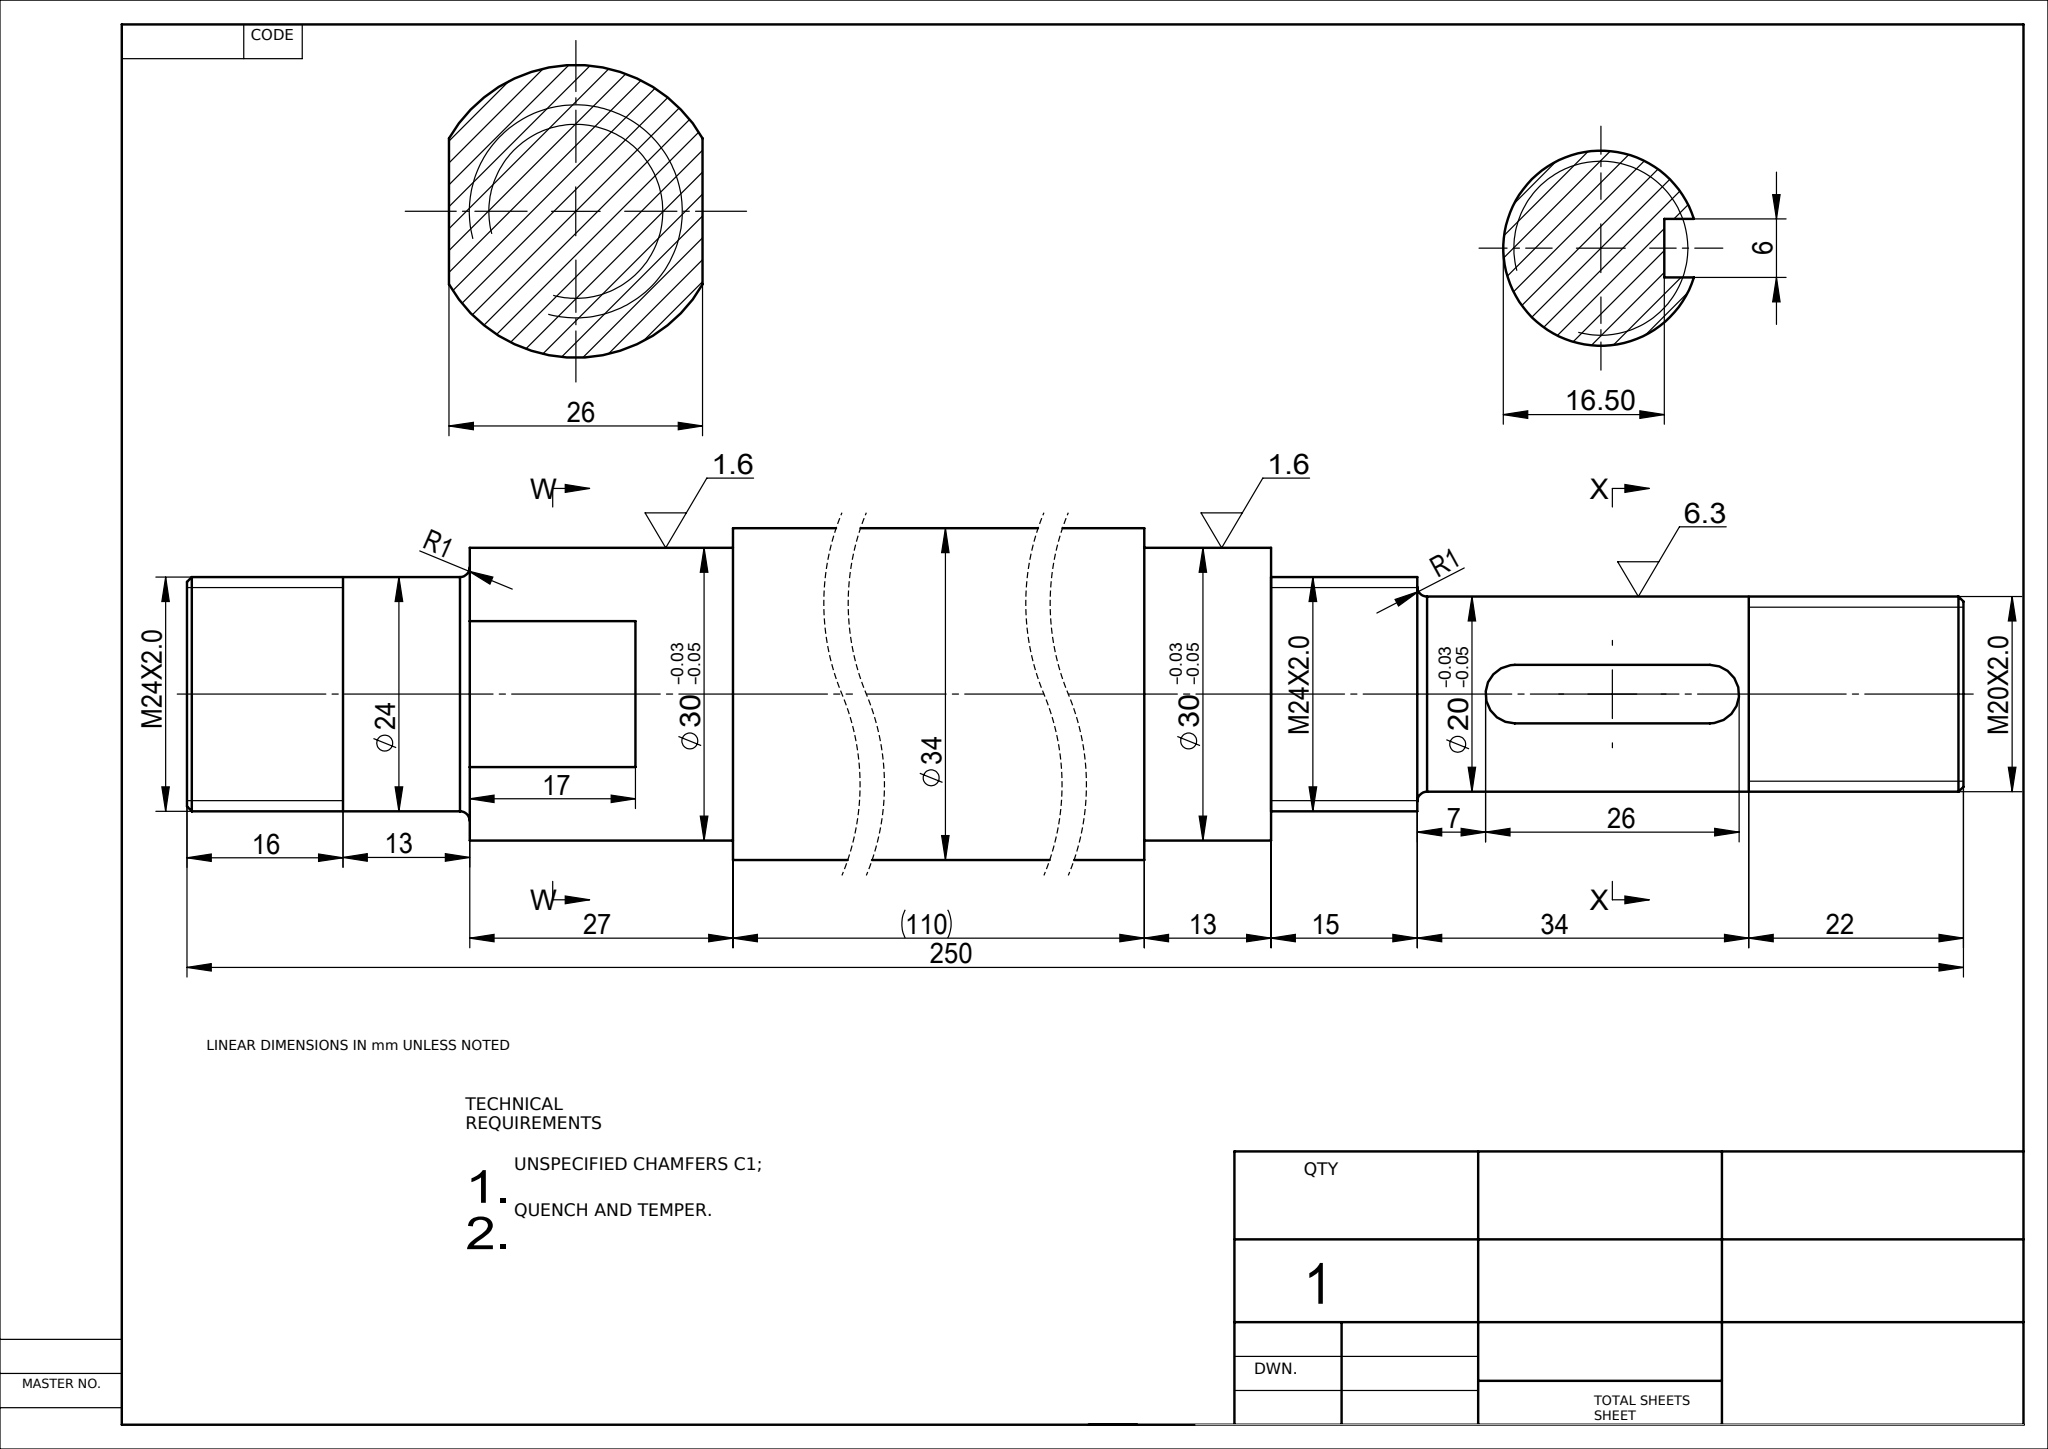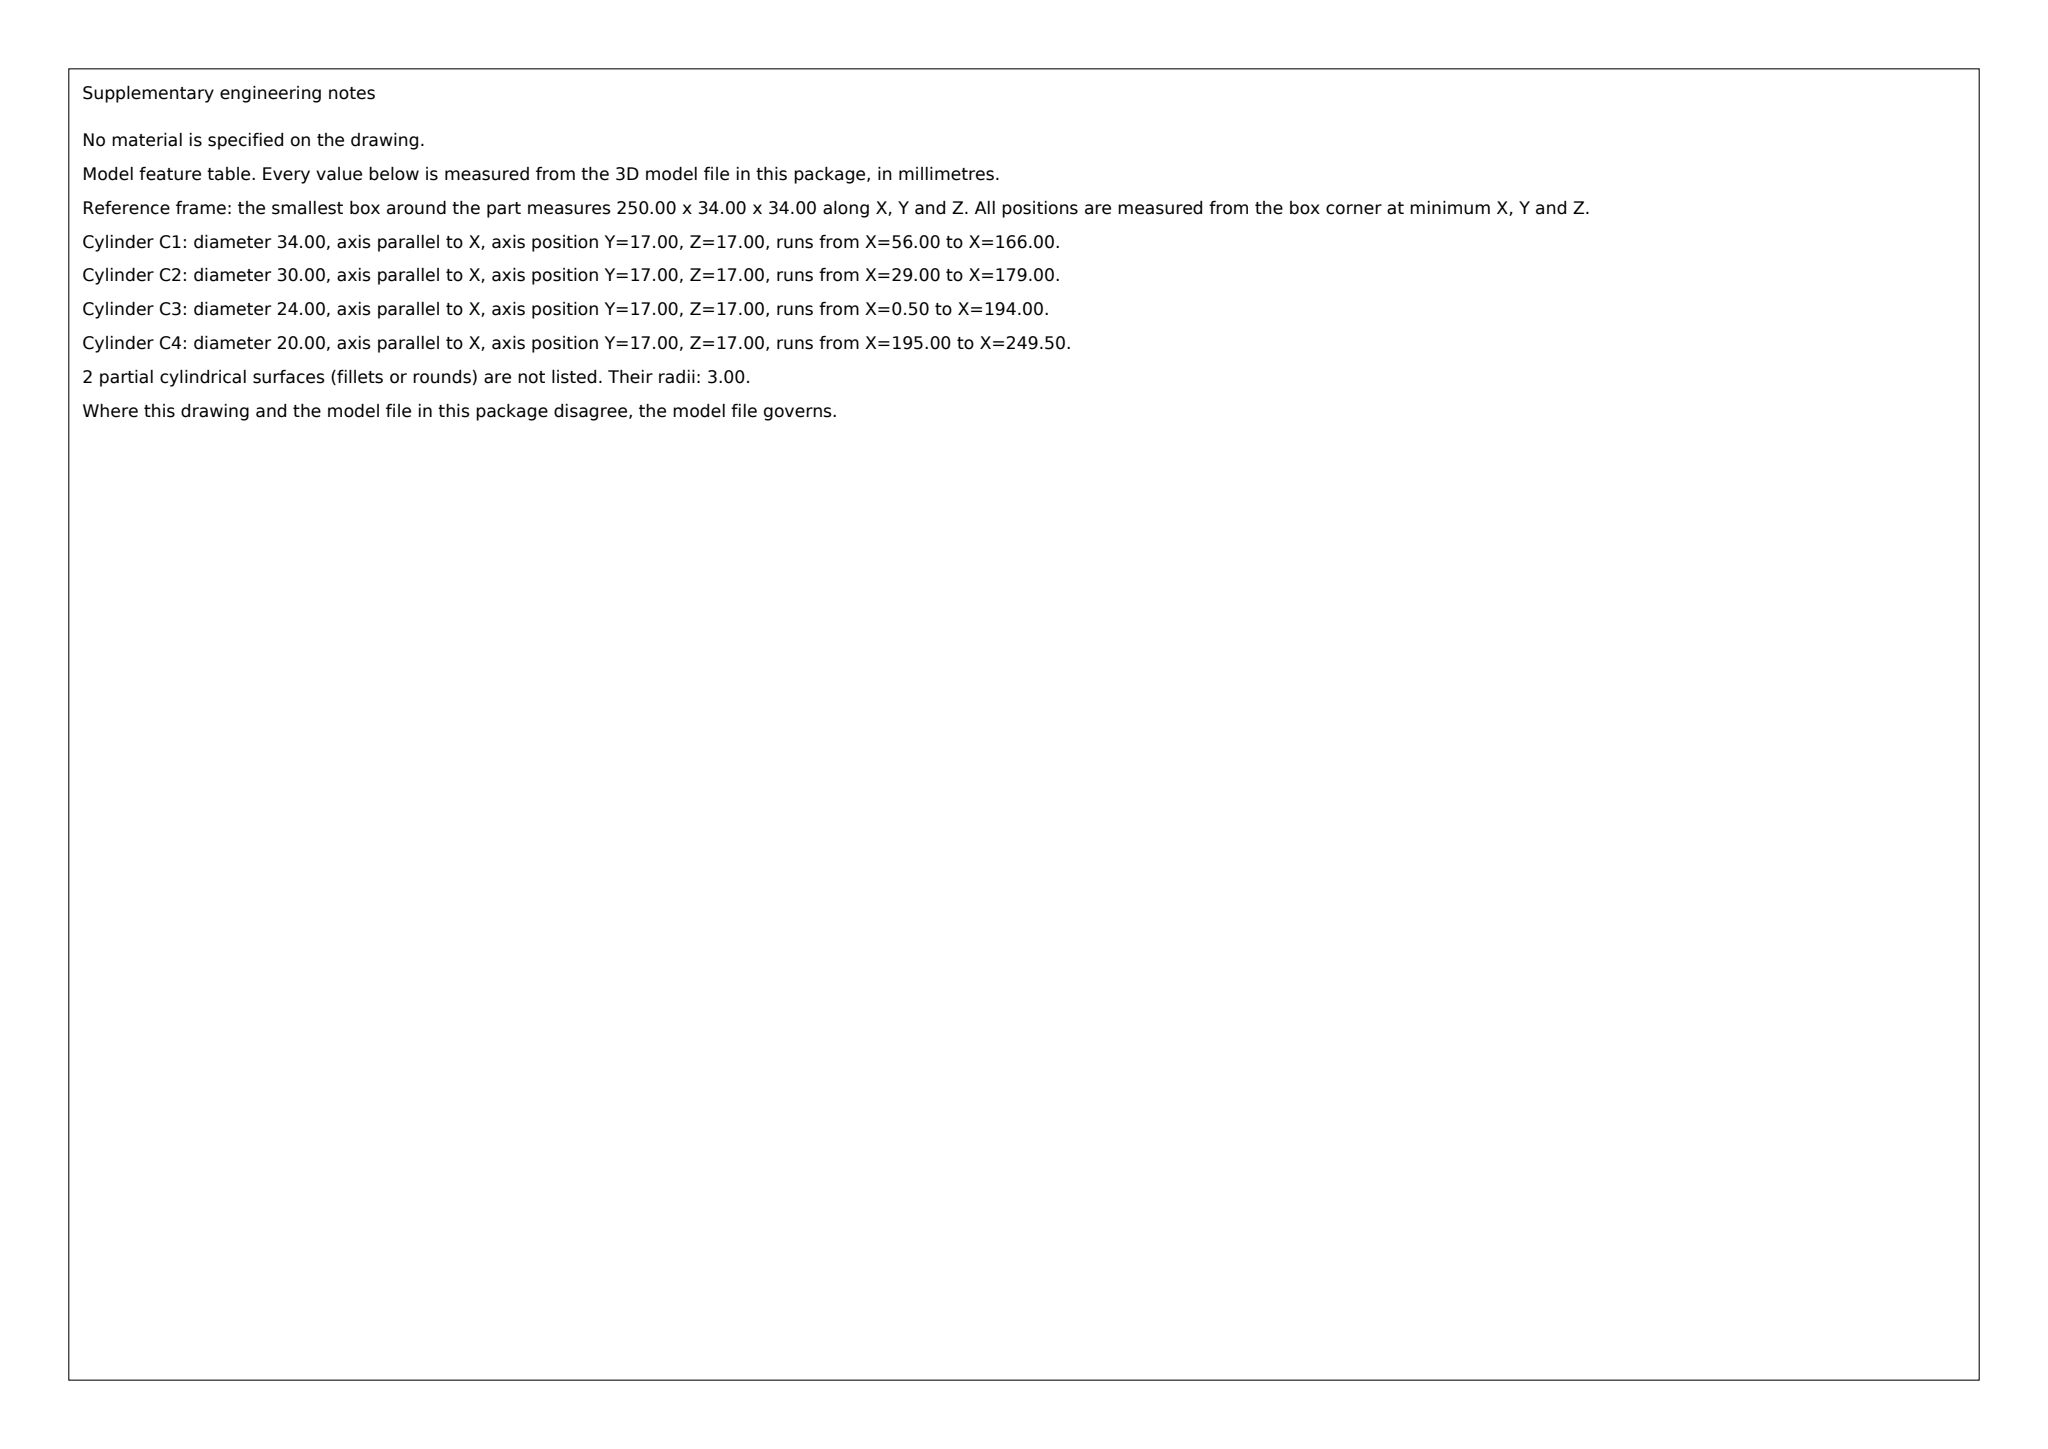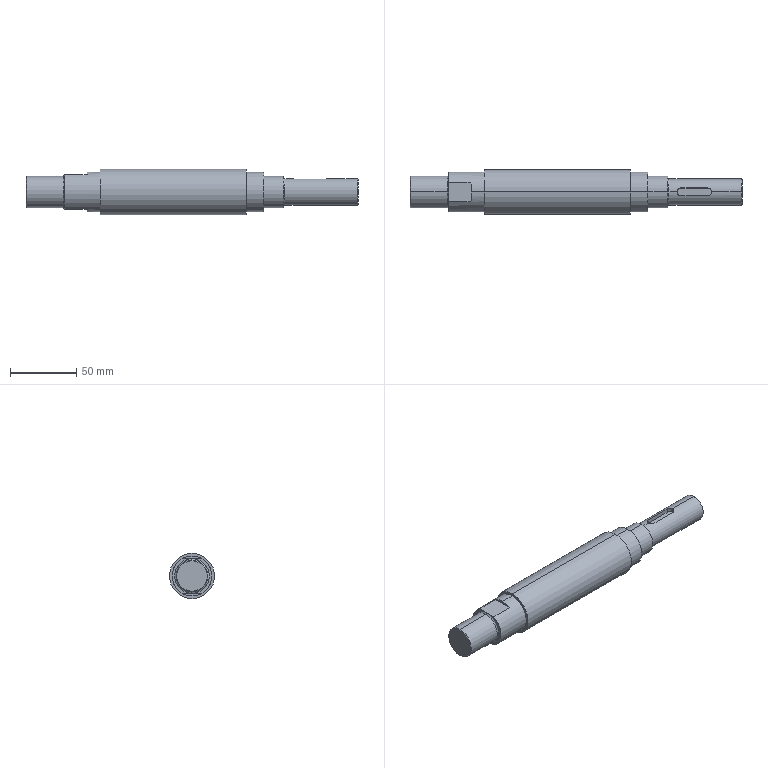Part | SolidWorks | mm | 1 solid | 38 faces | box 250 x 34 x 34 mm | volume 164471 mm3 | cylinder 15 | plane 15 | cone 4 | torus 4 | commonest cylinder face diameters 24 x4 30 x4 6 x3 20 x2 34 x2